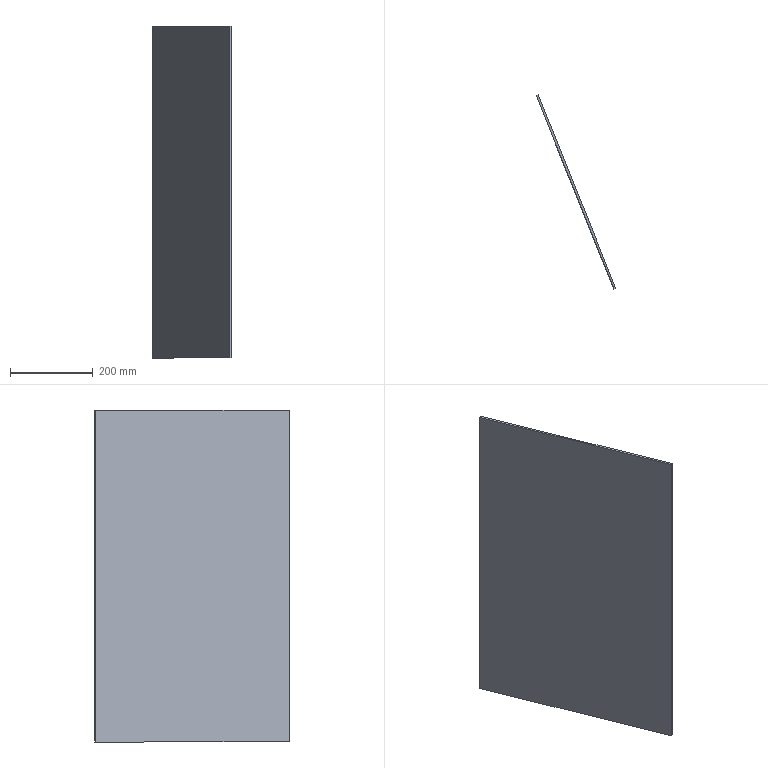Component | SolidWorks | GuardDoor-1_503.5-801-5-1 | 1 solid | 6 faces | box 191.99 x 469.21 x 801 mm | volume 2016517 mm3 | plane 6
build123d program:
from build123d import *

# Parameters (mm, degrees)
SKETCH1_W           = 503.5
SKETCH1_H           = 801
BOSS_EXTRUDE1_DEPTH = 5


with BuildPart() as part:
    # Sketch1 → Boss-Extrude1 (new body)
    with BuildSketch(Plane.XY):
        with Locations((251.75, -400.5)):
            Rectangle(SKETCH1_W, SKETCH1_H)
    extrude(amount=BOSS_EXTRUDE1_DEPTH)


solid = part.part

# Placed as in the assembly
solid = solid.moved(Location((1065.732, 675.72, -400.5), (90, -68.155, -180)))
STEP:
#1=CARTESIAN_POINT('',(41.775,26.53,15.768));
#2=VERTEX_POINT('',#1);
#3=CARTESIAN_POINT('',(41.775,26.53,-15.768));
#4=VERTEX_POINT('',#3);
#5=CARTESIAN_POINT('',(41.775,26.53,15.768));
#6=DIRECTION('',(0.,0.,-1.));
#7=VECTOR('',#6,39.37);
#8=LINE('',#5,#7);
#9=EDGE_CURVE('',#2,#4,#8,.T.);
#10=ORIENTED_EDGE('',*,*,#9,.T.);
#11=CARTESIAN_POINT('',(41.958,26.603,-15.768));
#12=VERTEX_POINT('',#11);
#13=CARTESIAN_POINT('',(41.958,26.603,-15.768));
#14=DIRECTION('',(-0.9282,-0.3721,-0.));
#15=VECTOR('',#14,39.37);
#16=LINE('',#13,#15);
#17=EDGE_CURVE('',#12,#4,#16,.T.);
#18=ORIENTED_EDGE('',*,*,#17,.F.);
#19=CARTESIAN_POINT('',(41.958,26.603,15.768));
#20=VERTEX_POINT('',#19);
#21=CARTESIAN_POINT('',(41.958,26.603,15.768));
#22=DIRECTION('',(0.,0.,-1.));
#23=VECTOR('',#22,39.37);
#24=LINE('',#21,#23);
#25=EDGE_CURVE('',#20,#12,#24,.T.);
#26=ORIENTED_EDGE('',*,*,#25,.F.);
#27=CARTESIAN_POINT('',(41.958,26.603,15.768));
#28=DIRECTION('',(-0.9282,-0.3721,-0.));
#29=VECTOR('',#28,39.37);
#30=LINE('',#27,#29);
#31=EDGE_CURVE('',#20,#2,#30,.T.);
#32=ORIENTED_EDGE('',*,*,#31,.T.);
#33=EDGE_LOOP('',(#10,#18,#26,#32));
#34=FACE_OUTER_BOUND('',#33,.T.);
#35=CARTESIAN_POINT('',(41.958,26.603,15.768));
#36=DIRECTION('',(-0.3721,0.9282,-0.));
#37=DIRECTION('',(-0.,-0.,1.));
#38=AXIS2_PLACEMENT_3D('',#35,#36,#37);
#39=PLANE('',#38);
#40=ADVANCED_FACE('',(#34),#39,.F.);
#41=CARTESIAN_POINT('',(34.399,44.929,-15.768));
#42=VERTEX_POINT('',#41);
#43=CARTESIAN_POINT('',(41.775,26.53,-15.768));
#44=DIRECTION('',(-0.3721,0.9282,-0.));
#45=VECTOR('',#44,39.37);
#46=LINE('',#43,#45);
#47=EDGE_CURVE('',#4,#42,#46,.T.);
#48=ORIENTED_EDGE('',*,*,#47,.T.);
#49=CARTESIAN_POINT('',(34.582,45.003,-15.768));
#50=VERTEX_POINT('',#49);
#51=CARTESIAN_POINT('',(34.582,45.003,-15.768));
#52=DIRECTION('',(-0.9282,-0.3721,-0.));
#53=VECTOR('',#52,39.37);
#54=LINE('',#51,#53);
#55=EDGE_CURVE('',#50,#42,#54,.T.);
#56=ORIENTED_EDGE('',*,*,#55,.F.);
#57=CARTESIAN_POINT('',(41.958,26.603,-15.768));
#58=DIRECTION('',(-0.3721,0.9282,-0.));
#59=VECTOR('',#58,39.37);
#60=LINE('',#57,#59);
#61=EDGE_CURVE('',#12,#50,#60,.T.);
#62=ORIENTED_EDGE('',*,*,#61,.F.);
#63=ORIENTED_EDGE('',*,*,#17,.T.);
#64=EDGE_LOOP('',(#48,#56,#62,#63));
#65=FACE_OUTER_BOUND('',#64,.T.);
#66=CARTESIAN_POINT('',(41.958,26.603,-15.768));
#67=DIRECTION('',(-0.,0.,1.));
#68=DIRECTION('',(0.9282,0.3721,0.));
#69=AXIS2_PLACEMENT_3D('',#66,#67,#68);
#70=PLANE('',#69);
#71=ADVANCED_FACE('',(#65),#70,.F.);
#72=CARTESIAN_POINT('',(34.399,44.929,15.768));
#73=VERTEX_POINT('',#72);
#74=CARTESIAN_POINT('',(34.399,44.929,15.768));
#75=DIRECTION('',(-0.,-0.,1.));
#76=VECTOR('',#75,39.37);
#77=LINE('',#74,#76);
#78=EDGE_CURVE('',#42,#73,#77,.T.);
#79=ORIENTED_EDGE('',*,*,#78,.T.);
#80=CARTESIAN_POINT('',(34.582,45.003,15.768));
#81=VERTEX_POINT('',#80);
#82=CARTESIAN_POINT('',(34.582,45.003,15.768));
#83=DIRECTION('',(-0.9282,-0.3721,-0.));
#84=VECTOR('',#83,39.37);
#85=LINE('',#82,#84);
#86=EDGE_CURVE('',#81,#73,#85,.T.);
#87=ORIENTED_EDGE('',*,*,#86,.F.);
#88=CARTESIAN_POINT('',(34.582,45.003,15.768));
#89=DIRECTION('',(-0.,-0.,1.));
#90=VECTOR('',#89,39.37);
#91=LINE('',#88,#90);
#92=EDGE_CURVE('',#50,#81,#91,.T.);
#93=ORIENTED_EDGE('',*,*,#92,.F.);
#94=ORIENTED_EDGE('',*,*,#55,.T.);
#95=EDGE_LOOP('',(#79,#87,#93,#94));
#96=FACE_OUTER_BOUND('',#95,.T.);
#97=CARTESIAN_POINT('',(34.582,45.003,15.768));
#98=DIRECTION('',(0.3721,-0.9282,0.));
#99=DIRECTION('',(0.,0.,-1.));
#100=AXIS2_PLACEMENT_3D('',#97,#98,#99);
#101=PLANE('',#100);
#102=ADVANCED_FACE('',(#96),#101,.F.);
#103=CARTESIAN_POINT('',(41.775,26.53,15.768));
#104=DIRECTION('',(0.3721,-0.9282,0.));
#105=VECTOR('',#104,39.37);
#106=LINE('',#103,#105);
#107=EDGE_CURVE('',#73,#2,#106,.T.);
#108=ORIENTED_EDGE('',*,*,#107,.T.);
#109=ORIENTED_EDGE('',*,*,#31,.F.);
#110=CARTESIAN_POINT('',(41.958,26.603,15.768));
#111=DIRECTION('',(0.3721,-0.9282,0.));
#112=VECTOR('',#111,39.37);
#113=LINE('',#110,#112);
#114=EDGE_CURVE('',#81,#20,#113,.T.);
#115=ORIENTED_EDGE('',*,*,#114,.F.);
#116=ORIENTED_EDGE('',*,*,#86,.T.);
#117=EDGE_LOOP('',(#108,#109,#115,#116));
#118=FACE_OUTER_BOUND('',#117,.T.);
#119=CARTESIAN_POINT('',(41.958,26.603,15.768));
#120=DIRECTION('',(0.,-0.,-1.));
#121=DIRECTION('',(-0.9282,-0.3721,-0.));
#122=AXIS2_PLACEMENT_3D('',#119,#120,#121);
#123=PLANE('',#122);
#124=ADVANCED_FACE('',(#118),#123,.F.);
#125=ORIENTED_EDGE('',*,*,#25,.T.);
#126=ORIENTED_EDGE('',*,*,#61,.T.);
#127=ORIENTED_EDGE('',*,*,#92,.T.);
#128=ORIENTED_EDGE('',*,*,#114,.T.);
#129=EDGE_LOOP('',(#125,#126,#127,#128));
#130=FACE_OUTER_BOUND('',#129,.T.);
#131=CARTESIAN_POINT('',(41.958,26.603,15.768));
#132=DIRECTION('',(0.9282,0.3721,0.));
#133=DIRECTION('',(-0.3721,0.9282,-0.));
#134=AXIS2_PLACEMENT_3D('',#131,#132,#133);
#135=PLANE('',#134);
#136=ADVANCED_FACE('',(#130),#135,.T.);
#137=ORIENTED_EDGE('',*,*,#9,.F.);
#138=ORIENTED_EDGE('',*,*,#107,.F.);
#139=ORIENTED_EDGE('',*,*,#78,.F.);
#140=ORIENTED_EDGE('',*,*,#47,.F.);
#141=EDGE_LOOP('',(#137,#138,#139,#140));
#142=FACE_OUTER_BOUND('',#141,.T.);
#143=CARTESIAN_POINT('',(41.775,26.53,15.768));
#144=DIRECTION('',(0.9282,0.3721,0.));
#145=DIRECTION('',(-0.3721,0.9282,-0.));
#146=AXIS2_PLACEMENT_3D('',#143,#144,#145);
#147=PLANE('',#146);
#148=ADVANCED_FACE('',(#142),#147,.F.);
#149=CLOSED_SHELL('',(#40,#71,#102,#124,#136,#148));
#150=MANIFOLD_SOLID_BREP('',#149);
#151=CARTESIAN_POINT('',(0.,0.,0.));
#152=DIRECTION('',(0.,0.,1.));
#153=DIRECTION('',(1.,0.,0.));
#154=AXIS2_PLACEMENT_3D('',#151,#152,#153);
#155=(LENGTH_UNIT()NAMED_UNIT(*)SI_UNIT($,.METRE.));
#156=LENGTH_MEASURE_WITH_UNIT(LENGTH_MEASURE(0.0254),#155);
#157=DIMENSIONAL_EXPONENTS(1.,0.,0.,0.,0.,0.,0.);
#158=(CONVERSION_BASED_UNIT('',#156)LENGTH_UNIT()NAMED_UNIT(#157));
#159=UNCERTAINTY_MEASURE_WITH_UNIT(LENGTH_MEASURE(0.00001),#158,'','');
#160=(NAMED_UNIT(*)PLANE_ANGLE_UNIT()SI_UNIT($,.RADIAN.));
#161=(NAMED_UNIT(*)SI_UNIT($,.STERADIAN.)SOLID_ANGLE_UNIT());
#162=(GEOMETRIC_REPRESENTATION_CONTEXT(3)GLOBAL_UNCERTAINTY_ASSIGNED_CONTEXT((#159))GLOBAL_UNIT_ASSIGNED_CONTEXT((#158,#160,#161))REPRESENTATION_CONTEXT('',''));
#163=ADVANCED_BREP_SHAPE_REPRESENTATION('',(#150,#154),#162);
#164=COLOUR_RGB('',0.7922,0.8196,0.9333);
#165=FILL_AREA_STYLE_COLOUR('',#164);
#166=FILL_AREA_STYLE('',(#165));
#167=SURFACE_STYLE_FILL_AREA(#166);
#168=SURFACE_SIDE_STYLE('',(#167));
#169=SURFACE_STYLE_USAGE(.BOTH.,#168);
#170=PRESENTATION_STYLE_ASSIGNMENT((#169));
#171=STYLED_ITEM('',(#170),#150);
#172=PRESENTATION_LAYER_ASSIGNMENT('','',(#171));
#173=(LENGTH_UNIT()NAMED_UNIT(*)SI_UNIT($,.METRE.));
#174=LENGTH_MEASURE_WITH_UNIT(LENGTH_MEASURE(0.0254),#173);
#175=DIMENSIONAL_EXPONENTS(1.,0.,0.,0.,0.,0.,0.);
#176=(CONVERSION_BASED_UNIT('',#174)LENGTH_UNIT()NAMED_UNIT(#175));
#177=UNCERTAINTY_MEASURE_WITH_UNIT(LENGTH_MEASURE(0.00001),#176,'','');
#178=(NAMED_UNIT(*)PLANE_ANGLE_UNIT()SI_UNIT($,.RADIAN.));
#179=(NAMED_UNIT(*)SI_UNIT($,.STERADIAN.)SOLID_ANGLE_UNIT());
#180=(GEOMETRIC_REPRESENTATION_CONTEXT(3)GLOBAL_UNCERTAINTY_ASSIGNED_CONTEXT((#177))GLOBAL_UNIT_ASSIGNED_CONTEXT((#176,#178,#179))REPRESENTATION_CONTEXT('',''));
#181=MECHANICAL_DESIGN_GEOMETRIC_PRESENTATION_REPRESENTATION('',(#171),#180);